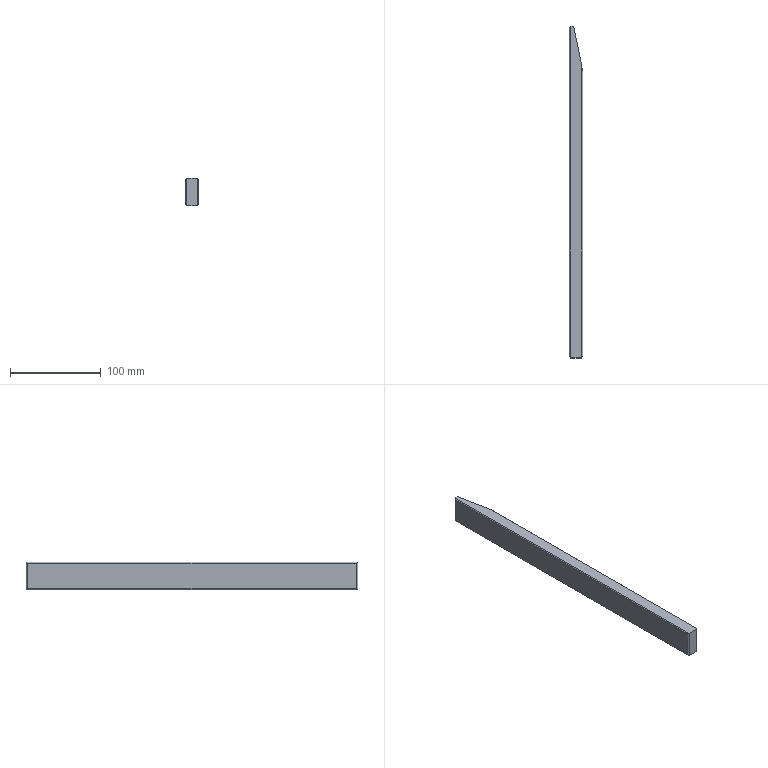Component | SolidWorks | AX00-100.1.1-1_AXFrame_A.1.1-1_09.1.1-1 | 1 solid | 14 faces | box 15 x 365 x 30 mm | volume 155893 mm3 | plane 14
build123d program:
from build123d import *

# Parameters (mm, degrees)
SKETCH1_W           = 365
SKETCH1_H           = 30
BOSS_EXTRUDE1_DEPTH = 7.5
CHAMFER1_SIZE       = 10
CHAMFER1_SIZE2      = 50
CHAMFER2_SIZE       = 2
CHAMFER3_SIZE       = 1


with BuildPart() as part:
    # Sketch1 → Boss-Extrude1 (new, symmetric)
    with BuildSketch(Plane.XY):
        Rectangle(SKETCH1_W, SKETCH1_H)
    extrude(amount=BOSS_EXTRUDE1_DEPTH, both=True)

    # Chamfer1
    chamfer1_edges = [part.edges().sort_by_distance(p)[0] for p in [
        (182.5, 0, 7.5),
    ]]
    chamfer1_side = [part.faces().sort_by_distance(p)[0] for p in [
        (182.5, 0, 0),
    ]]
    chamfer(chamfer1_edges, length=CHAMFER1_SIZE, length2=CHAMFER1_SIZE2, reference=chamfer1_side[0])

    # Chamfer2
    chamfer2_edges = [part.edges().sort_by_distance(p)[0] for p in [
        (-182.5, 0, 7.5),
        (-182.5, 0, -7.5),
        (182.5, 0, -7.5),
    ]]
    chamfer(chamfer2_edges, length=CHAMFER2_SIZE)

    # Chamfer3
    chamfer3_edges = [part.edges().sort_by_distance(p)[0] for p in [
        (-24, 15, 7.5),
        (0, 15, -7.5),
        (0, -15, -7.5),
        (-24, -15, 7.5),
    ]]
    chamfer(chamfer3_edges, length=CHAMFER3_SIZE)


solid = part.part

# Placed as in the assembly
solid = solid.moved(Location((-83.869, 1330.864, 167.5), (90, 90, 0)))